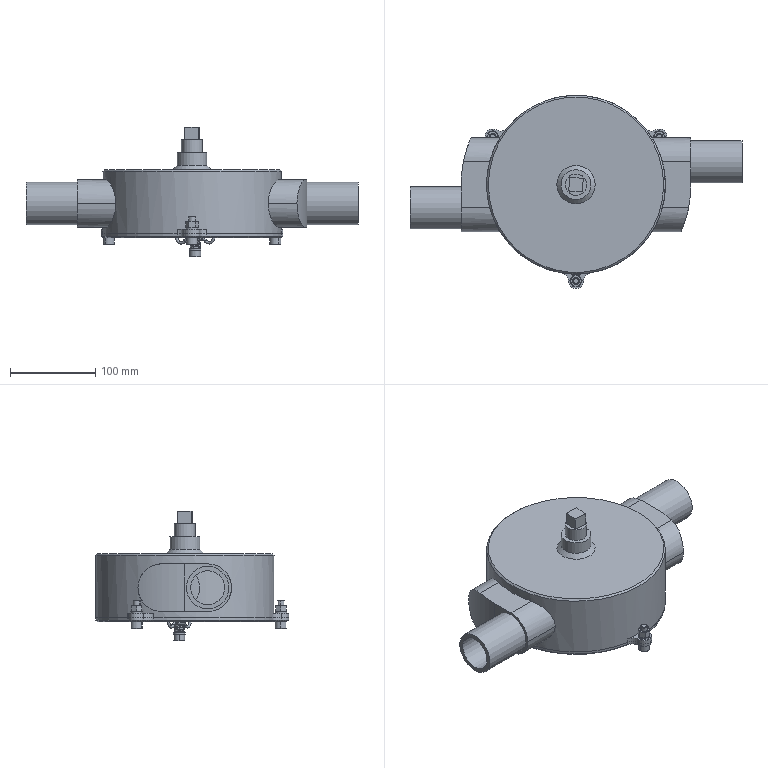Assembly | NX | mm | 23 component files | 23 solids | 448 faces | box 390 x 227 x 152.6 mm | volume 2398358 mm3 | plane 183 | cylinder 155 | cone 74 | torus 25 | spline 11 | commonest cylinder face diameters 8 x16 50 x14 8.88 x12 13.68 x12 20 x12 3 x10 200 x8 56 x8
Bill of materials:
unnamed part 1 | 1 |  | Shallow round box-like body with two tubular spigots coming out on opposite sides, a small hollow boss in the middle of the top face, and small tabs with holes around the base.
unnamed part 2 | 1 |  | Bent round-wire or rod part with a closed ring eye in the middle and two straight arms going opposite ways, each ending in a U-shaped hook bend.
unnamed part 3 | 1 |  | Thin, flat, circular plate with three lugs with holes around the edge, and a raised stepped cylindrical boss in the centre holding a non-circular through-opening.
unnamed part 4 | 4 |  | Headed pin or bolt-like part: a short cylindrical head of larger diameter and a long, smooth cylindrical shank with a chamfered end.
unnamed part 5 | 4 |  | Flat split ring: an annulus of constant rectangular cross-section with one radial cut through the ring.
unnamed part 6 | 1 |  | Helical coil spring form of round wire with several closely spaced turns and flattened (ground-like) end faces.
unnamed part 7 | 1 |  | Flat cylindrical disc head with a single smaller cylindrical stem on its axis, giving a T-shaped profile; the stem end has a small angled cut or flat.
unnamed part 8 | 3 |  | Hexagonal nut-shaped body with a plain cylindrical through-bore and chamfered corners at both faces.
unnamed part 9 | 1 |  | Short cylindrical hub with several radial through-holes around its side wall and a stepped central pin on top whose tip has a V/notched or flatted profile.
unnamed part 10 | 6 |  | Thick cylindrical disc with a conical central recess, from which a slender rod sticks out and ends in a perpendicular cylindrical crossbar, giving a T-handle-like rod on a disc.
Mates:
1. fix | Pump_Body 1 component
2. concentric | Pump_Cover 1 arc | Pump_Body 1 edge
3. concentric | Pump_Cover 1 arc | Pump_Body 1 edge
4. touch align | Rotor 1 face | Pump_Body 1 face
5. center | Rotor 1 face | Rotor 1 face | Pump_Body 1 face | Pump_Body 1 face
6. center | Connecting_Rod 1 face | Connecting_Rod 1 face | Pump_Cover 1 face | Pump_Cover 1 face
7. touch align | Rotor 1 face | Connecting_Rod 1 face
8. touch align | Piston 6 face | Rotor 1 face
9. parallel | Piston 6 face | Pump_Body 1 face
10. touch align | Piston 6 face | Connecting_Rod 1 face
11. touch align | Piston 5 face | Rotor 1 face
12. parallel | Piston 5 face | Pump_Body 1 face
13. touch align | Piston 5 face | Connecting_Rod 1 face
14. touch align | Piston 4 face | Rotor 1 face
15. parallel | Piston 4 face | Pump_Body 1 face
16. touch align | Piston 4 face | Connecting_Rod 1 face
17. touch align | Piston 3 face | Rotor 1 face
18. parallel | Piston 3 face | Pump_Body 1 face
19. touch align | Piston 3 face | Connecting_Rod 1 face
20. touch align | Piston 2 face | Rotor 1 face
21. parallel | Piston 2 face | Pump_Body 1 face
22. touch align | Piston 2 face | Connecting_Rod 1 face
23. touch align | Piston 1 face | Rotor 1 face
24. parallel | Piston 1 face | Connecting_Rod 1 face
25. touch align | Piston 1 face | Connecting_Rod 1 face
26. concentric | Lifting_Ring 1 arc | Pump_Cover 1 edge
27. concentric | Lifting_Ring 1 edge | Pump_Cover 1 edge
28. touch align | Connecting_Rod 1 face | Lifting_Ring 1 face
29. touch align | SPRING_CYLINDER_COMPRESSION_1 1 datumaxis | Lifting_Ring 1 face
30. touch align | SPRING_CYLINDER_COMPRESSION_1 1 face | Lifting_Ring 1 face
31. touch align | Saddle_Spring_Washer_8 4 face | Lifting_Ring 1 face
32. touch align | SPRING_CYLINDER_COMPRESSION_1 1 face | Saddle_Spring_Washer_8 4 face
33. concentric | Hex_Socket_Screw_M8x25 4 edge | Saddle_Spring_Washer_8 4 edge
34. concentric | Hex_Socket_Screw_M8x25 3 edge | Pump_Cover 1 edge
35. concentric | Saddle_Spring_Washer_8 3 edge | Pump_Body 1 edge
36. concentric | Saddle_Spring_Washer_8 3 edge | Hex_Nut_M8 3
37. bond | Pump_Body 1 component | assembly component
38. bond | Hex_Socket_Screw_M8x25 3 component | assembly component
39. bond | Saddle_Spring_Washer_8 3 component | assembly component
40. bond | Hex_Nut_M8 3 component | assembly component
41. bond | Hex_Socket_Screw_M8x25 2 component | assembly component
42. bond | Saddle_Spring_Washer_8 2 component | assembly component
43. bond | Hex_Nut_M8 2 component | assembly component
44. bond | Hex_Socket_Screw_M8x25 1 component | assembly component
45. bond | Saddle_Spring_Washer_8 1 component | assembly component
46. bond | Hex_Nut_M8 1 component | assembly component
47. circular | assembly datumaxis | assembly cartesiancoordinatesystem | assembly cartesiancoordinatesystem | assembly cartesiancoordinatesystem
48. circular | assembly datumaxis | assembly cartesiancoordinatesystem | assembly cartesiancoordinatesystem | assembly cartesiancoordinatesystem
49. circular | assembly datumaxis | assembly cartesiancoordinatesystem | assembly cartesiancoordinatesystem | assembly cartesiancoordinatesystem